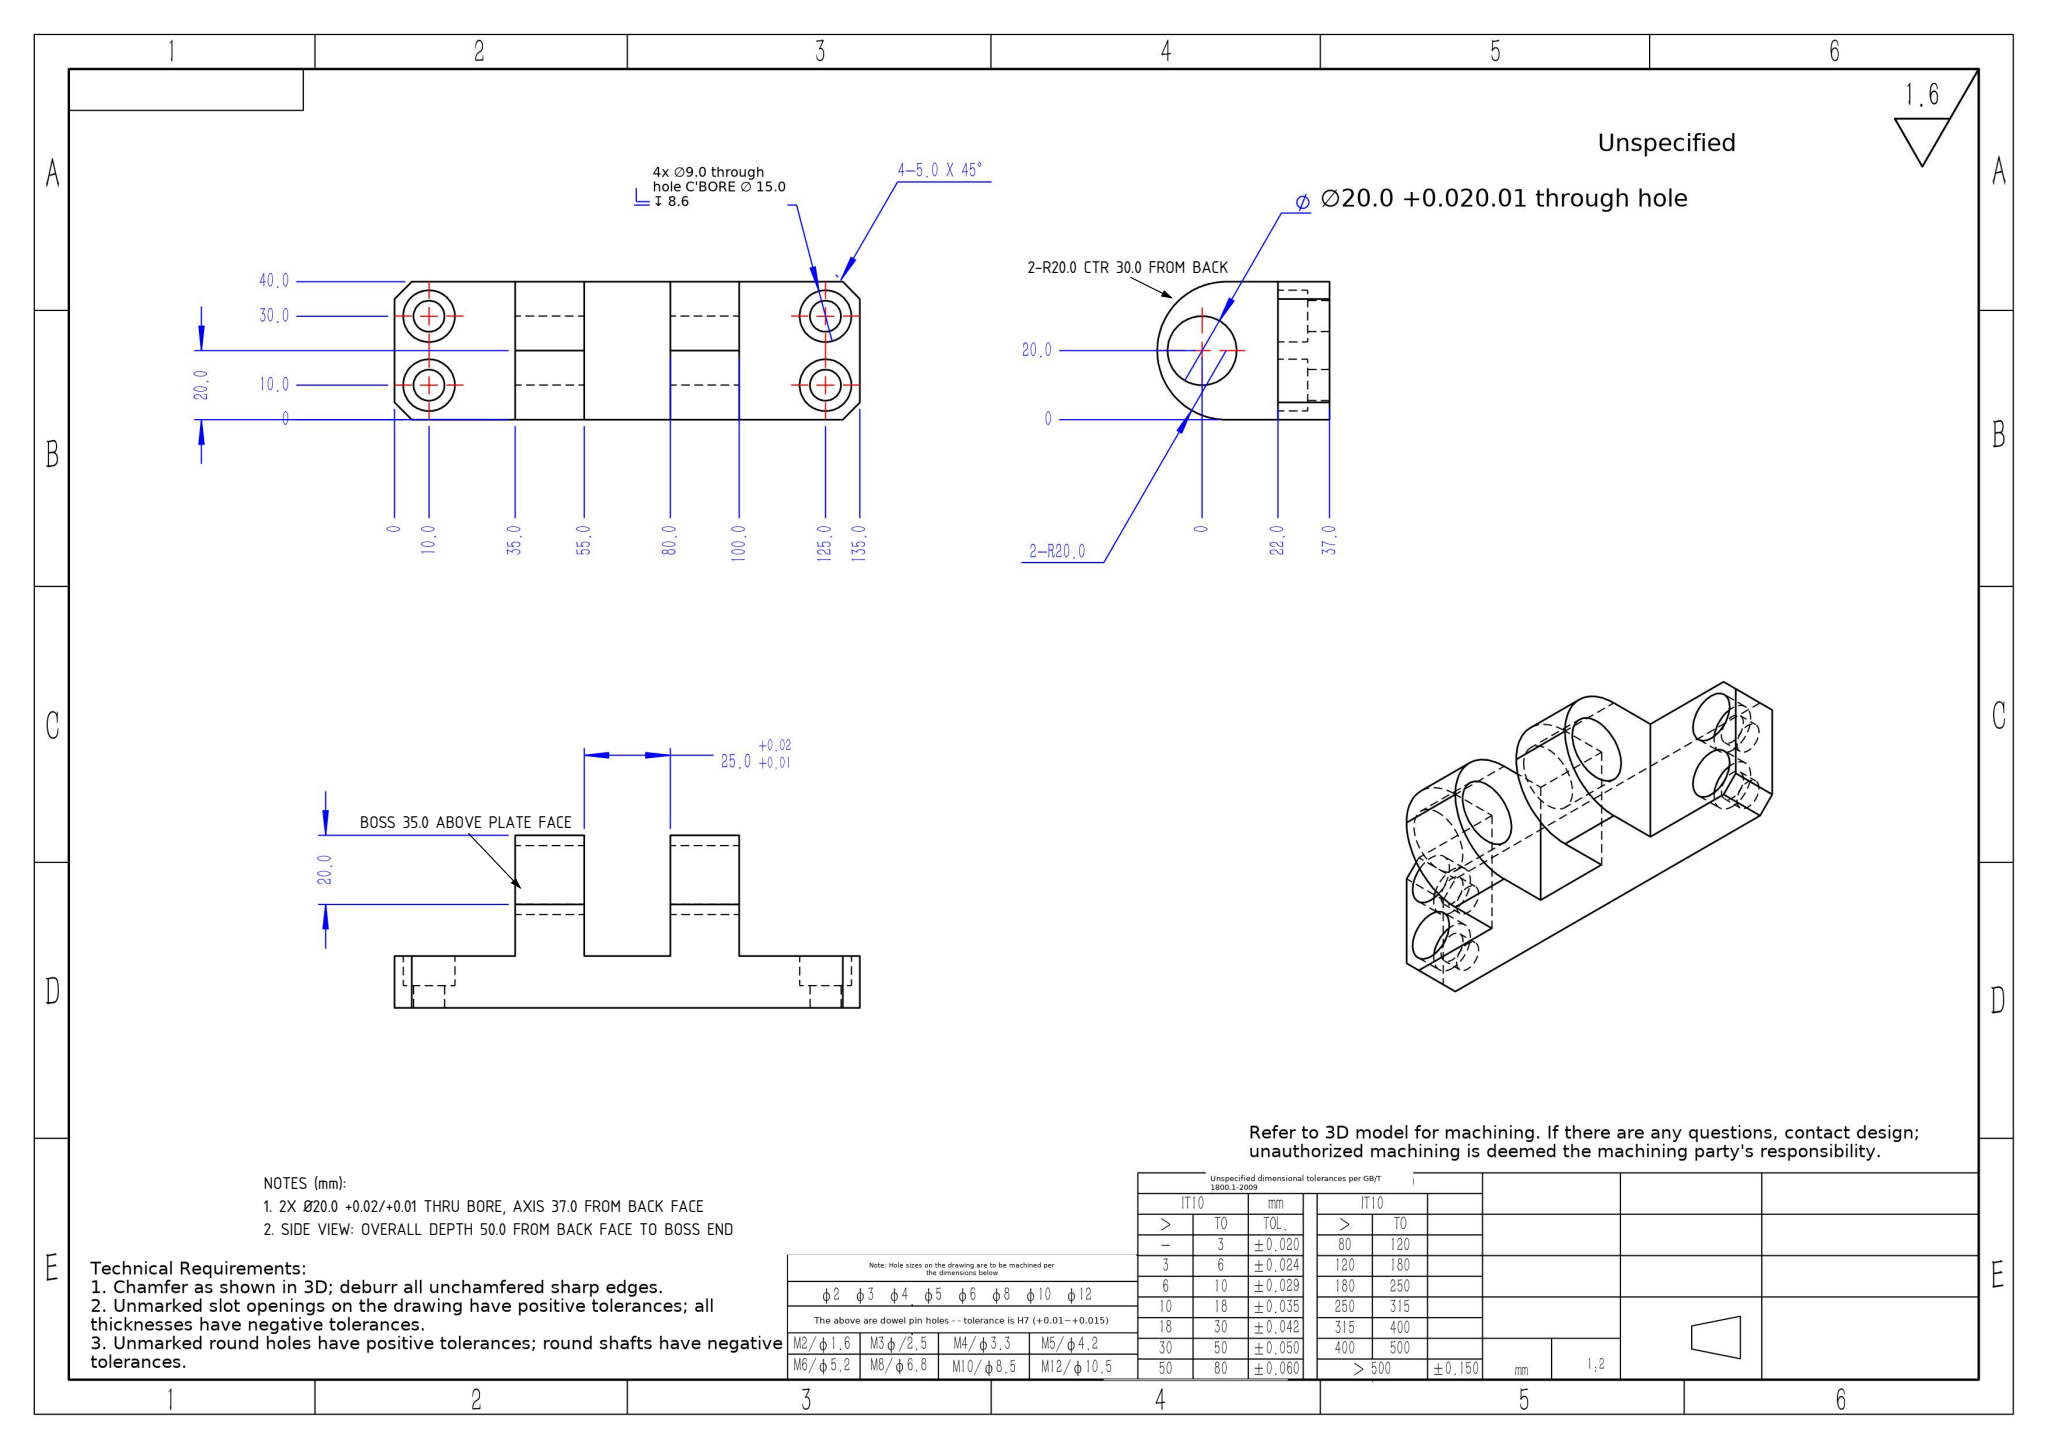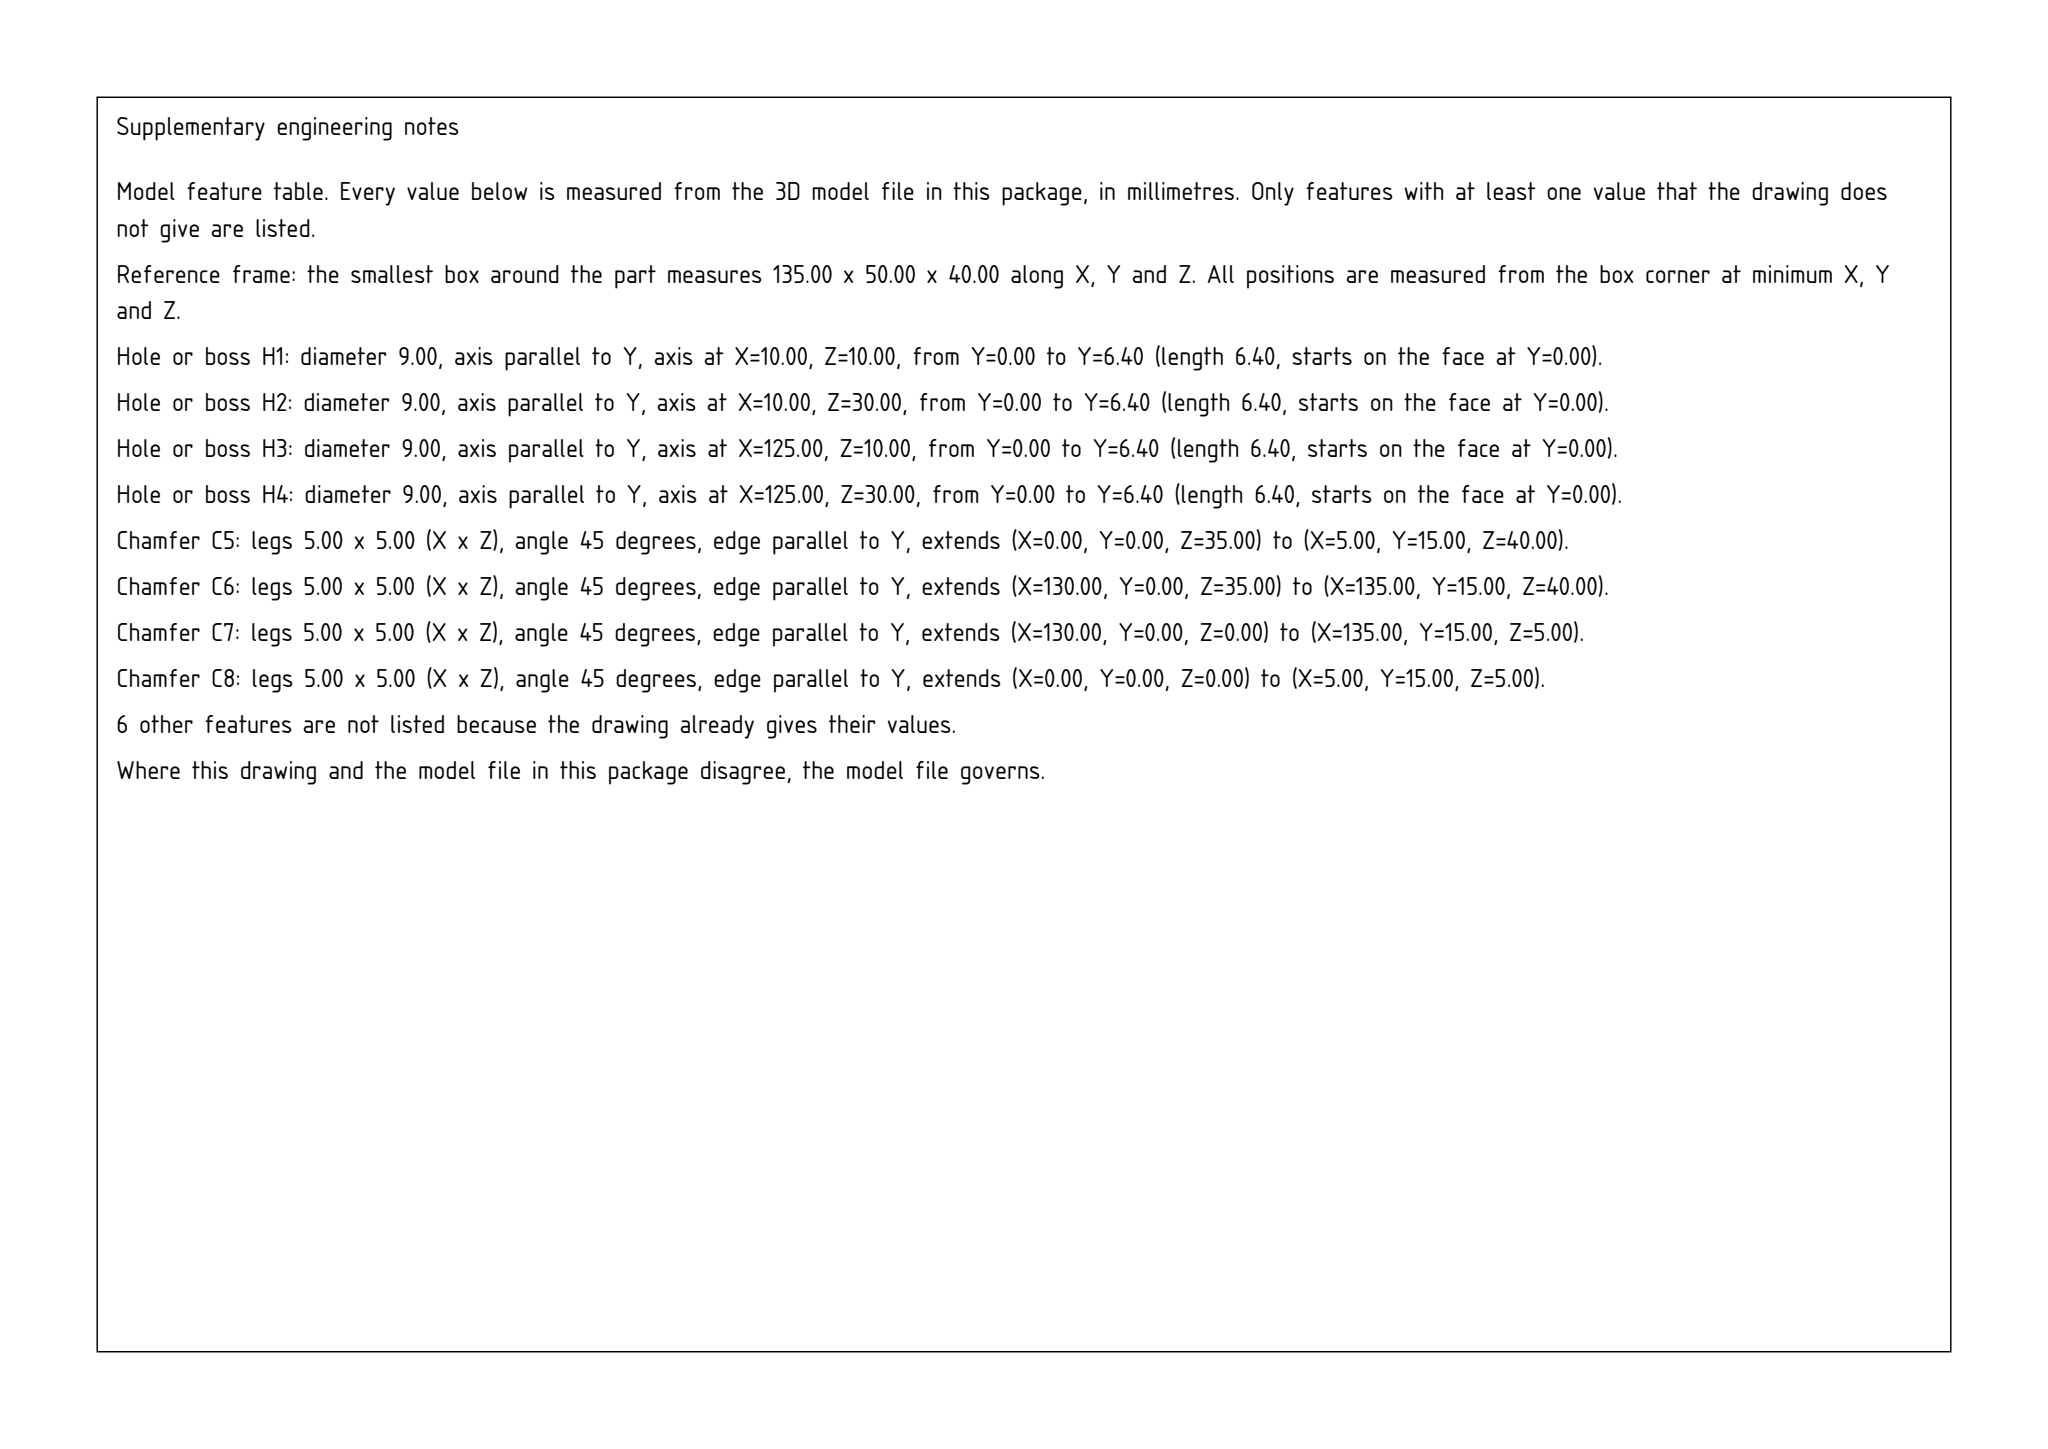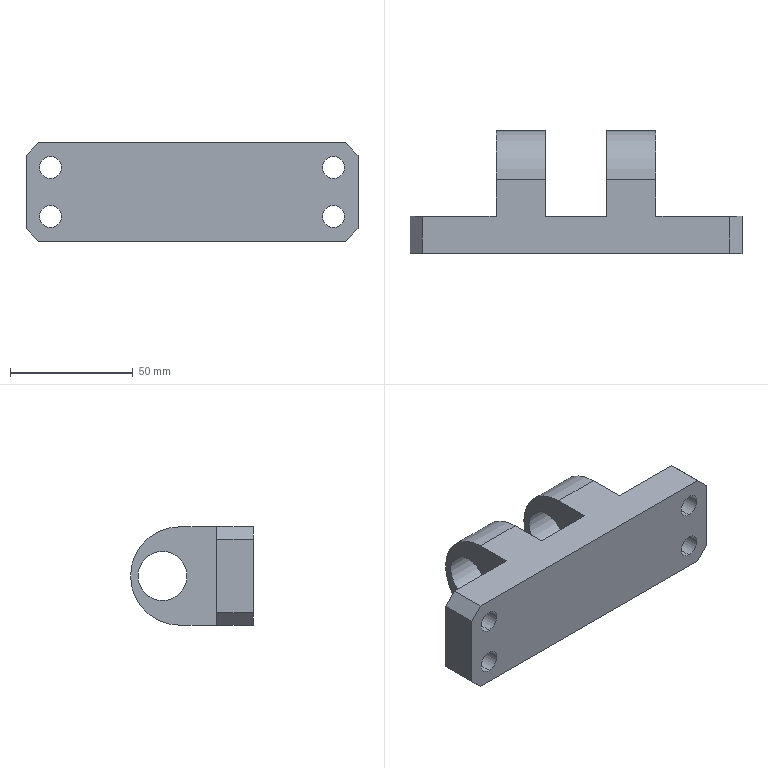Part | SolidWorks | mm | 1 solid | 44 faces | box 135 x 50 x 40 mm | volume 109109 mm3 | cylinder 24 | plane 20 | commonest cylinder face diameters 15 x8 9 x8 20 x4 40 x4
Drawing notes:
2X Ø20.0 +0.02/+0.01 THRU BORE, AXIS 37.0 FROM BACK FACE | from the solid: cylinders: hole/bore dia 20.0 axis x at (y=37.0, z=20.0), x 35-55 and 80-100, 360 deg, thru both bosses
SIDE VIEW: OVERALL DEPTH 50.0 FROM BACK FACE TO BOSS END | from the solid: bbox y 0->50; back face plane y=0, boss outer extent y=50
2-R20.0 CTRS 30.0 FROM BACK FACE, 7.0 BEHIND Ø20 BORE AXIS | from the solid: R20 arcs axis_pos y=30.0; Ø20 bore axis y=37.0; 37-30=7
BOSS PROJECTS 35.0 FROM 15.0 PLATE FACE (Y=15 TO Y=50) | from the solid: plate face plane y=15.0; boss end y=50.0